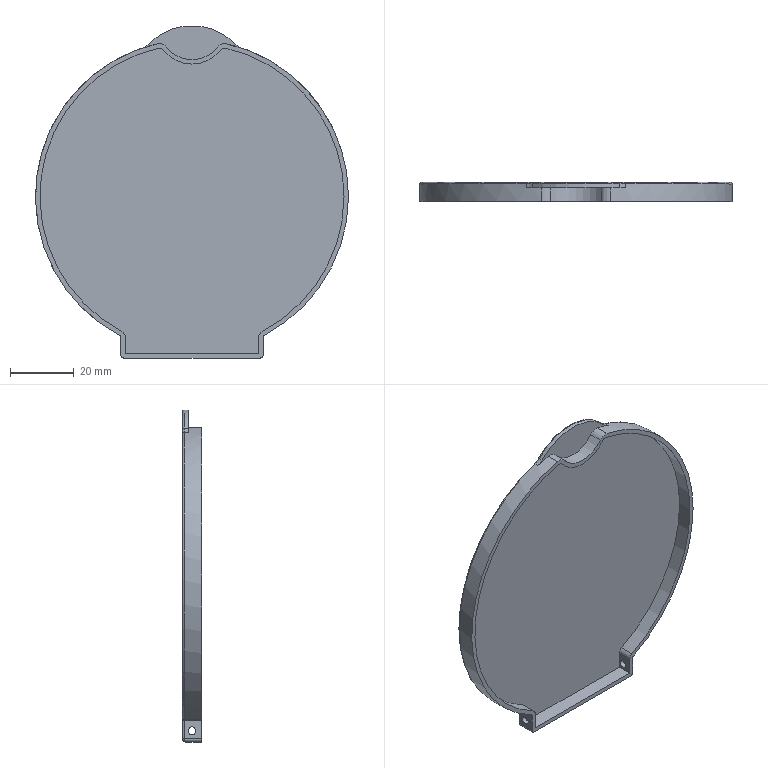Component | SolidWorks | WuliangyeBottleCap-1-1 | 1 solid | 48 faces | volume 13070 mm3 | cylinder 28 | plane 10 | torus 8 | spline 2 | commonest cylinder face diameters 2.5 x4 1 x4 95.6 x3 98.4 x3 2 x3 10 x2 6 x2 3.2 x2